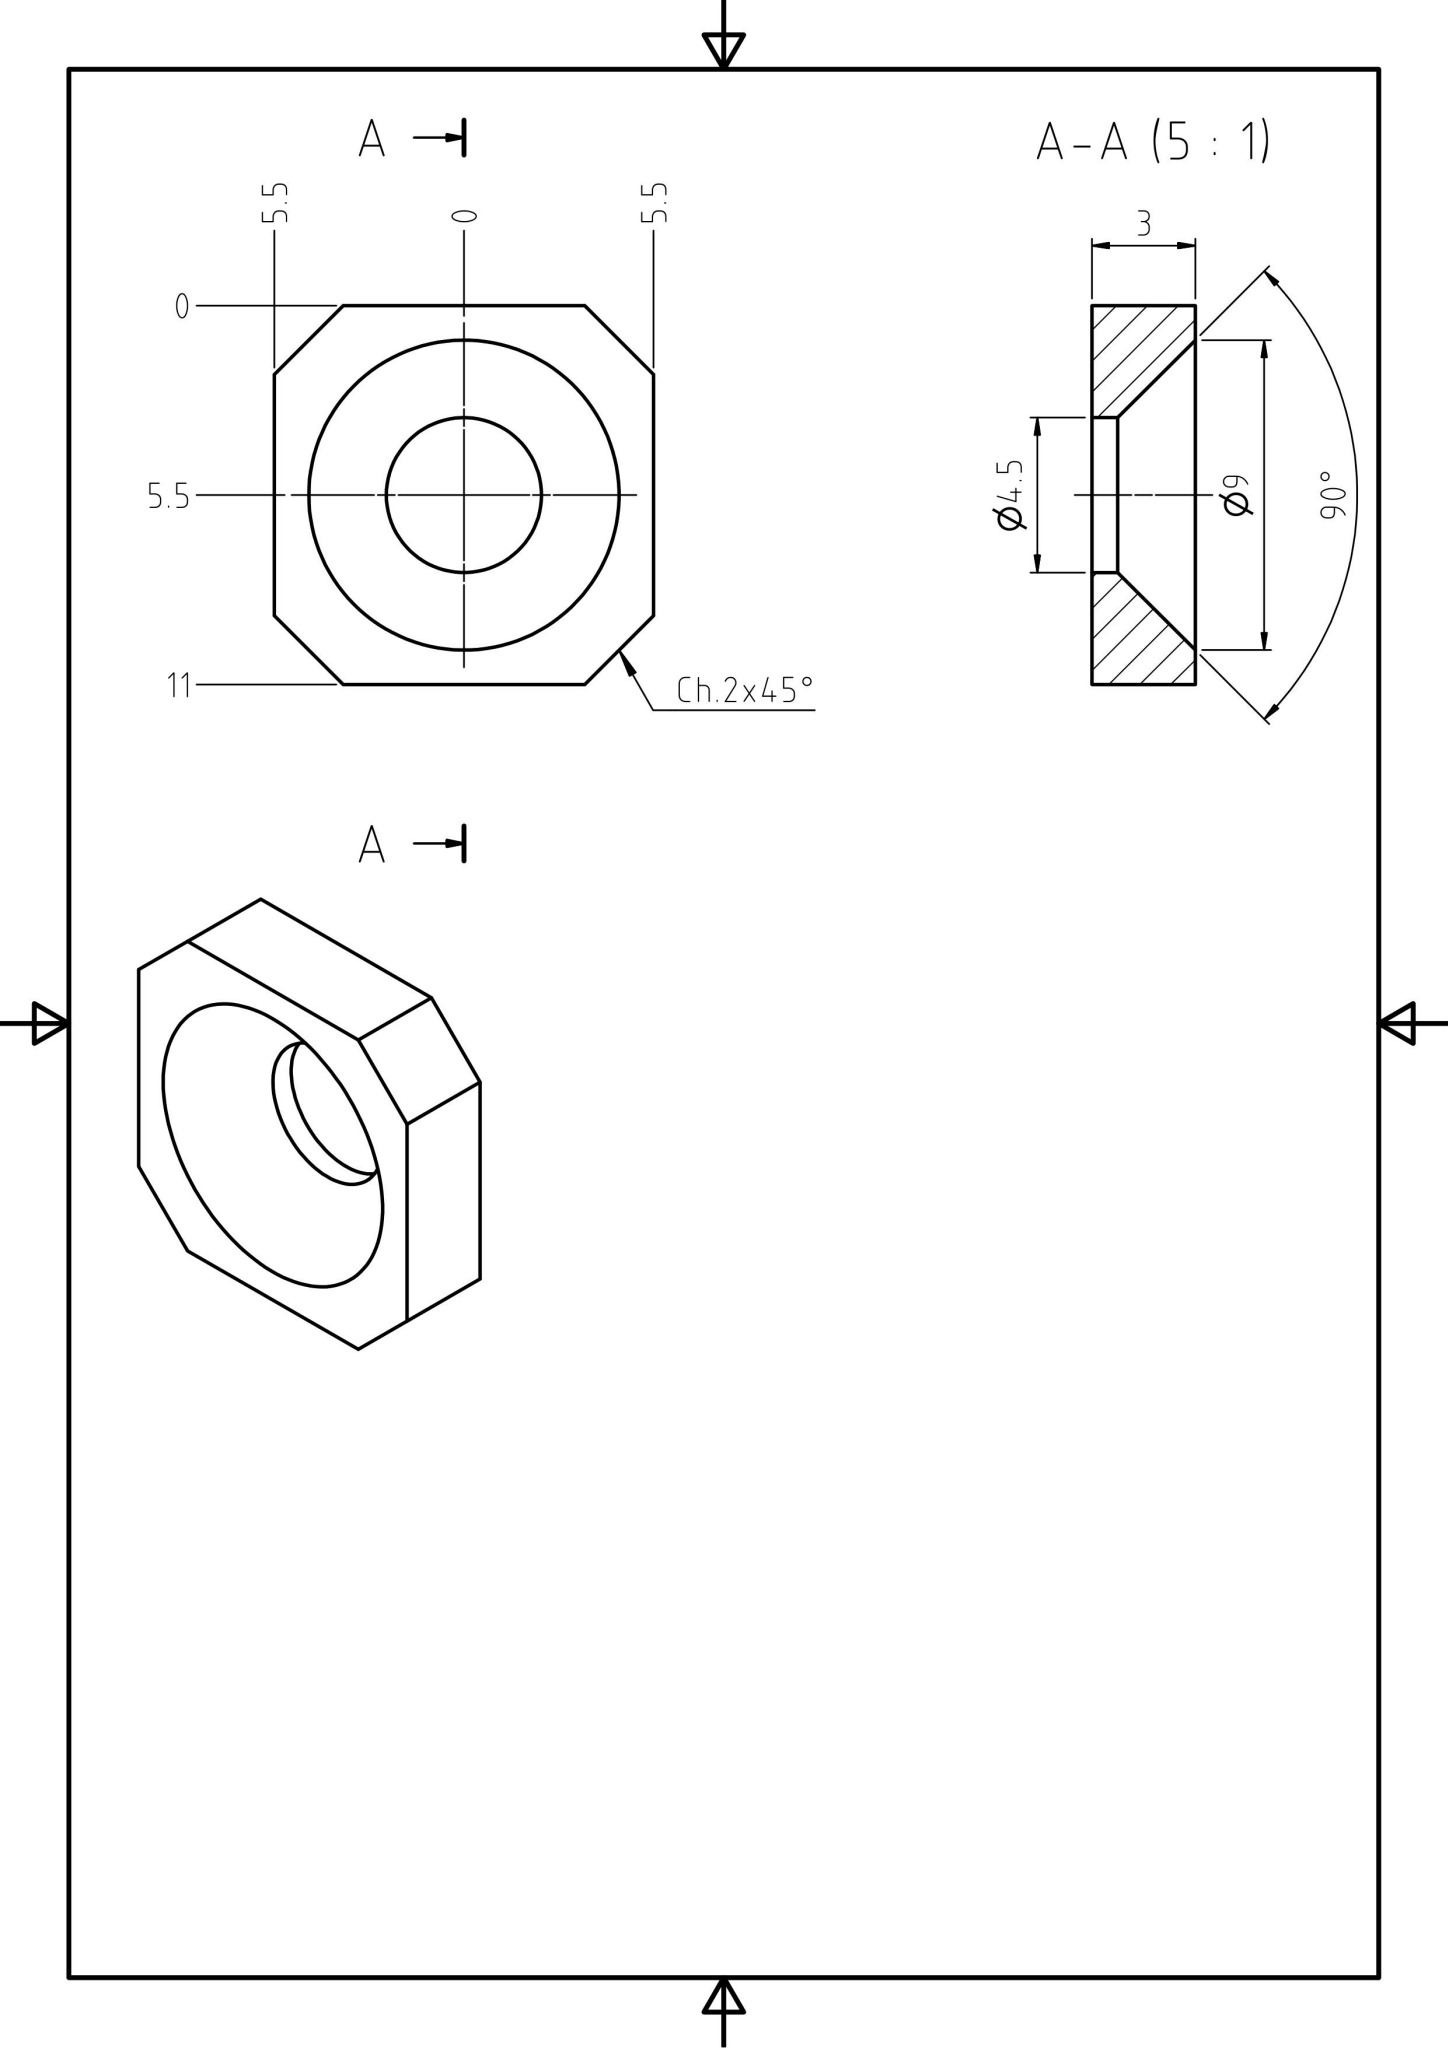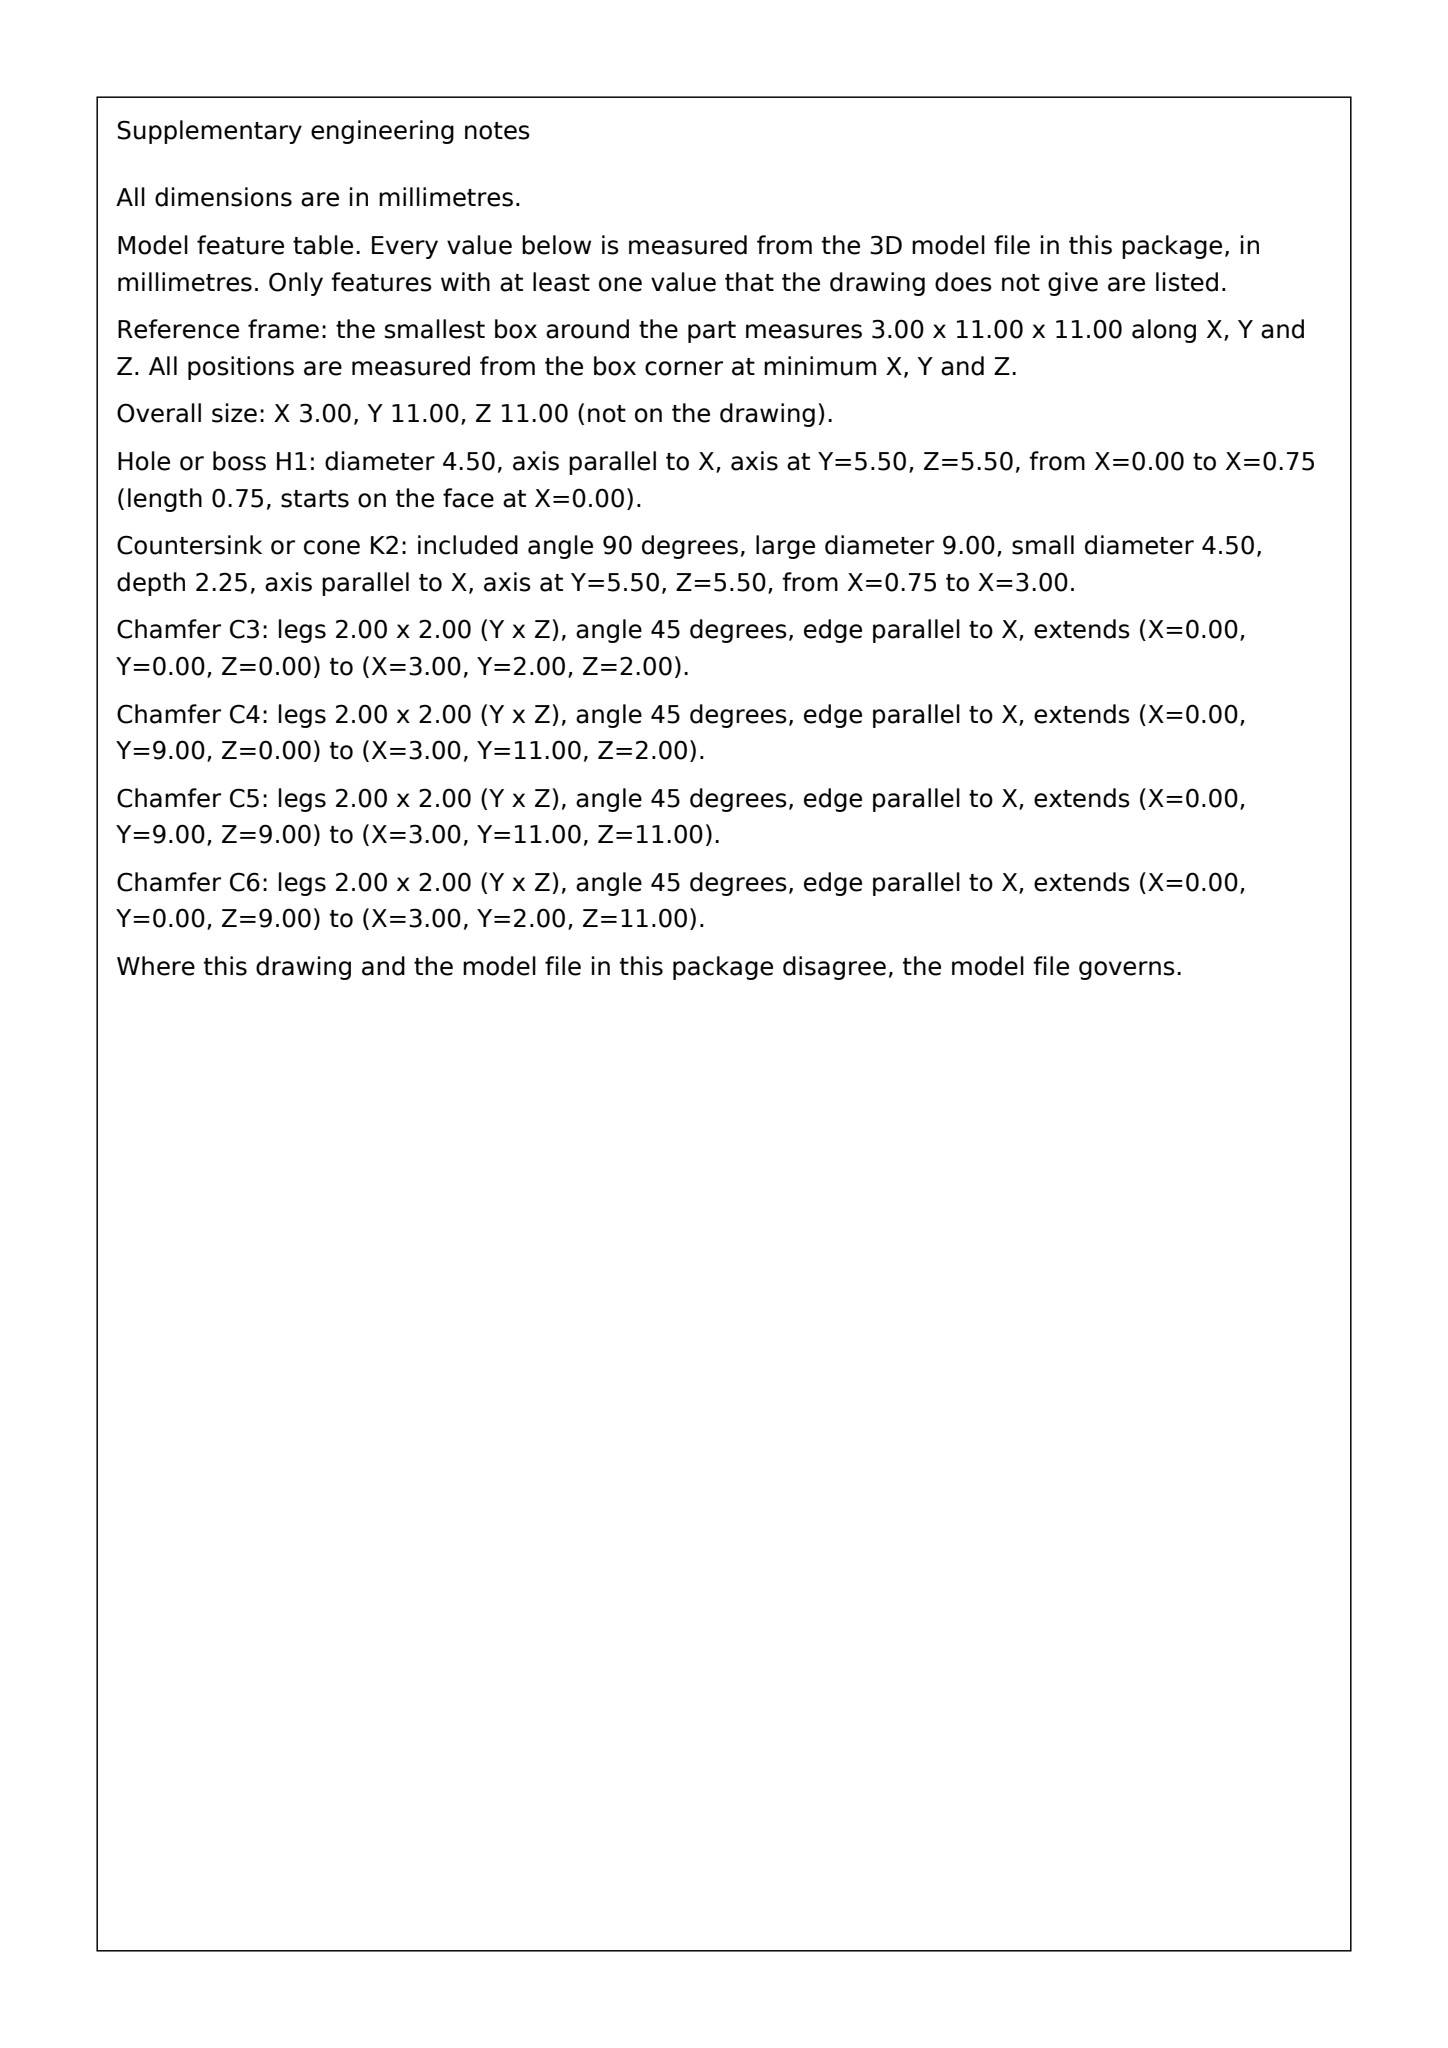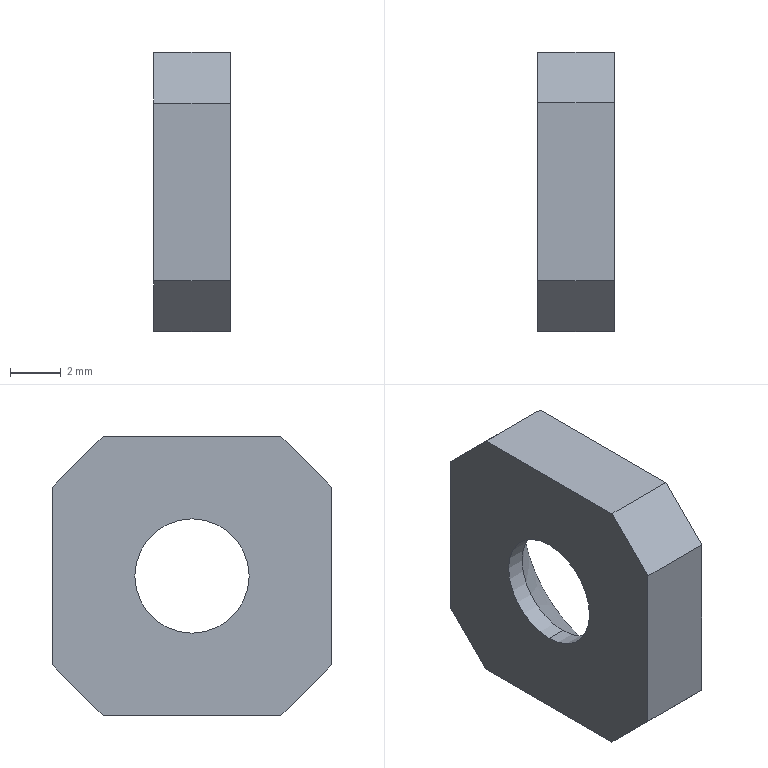Part | SolidWorks | mm | 1 solid | 14 faces | box 3 x 11 x 11 mm | volume 244 mm3 | plane 10 | cylinder 2 | cone 2 | commonest cylinder face diameters 4.5 x2
STEP:
#1=CARTESIAN_POINT('',(0.,0.,2.25));
#2=VERTEX_POINT('',#1);
#3=CARTESIAN_POINT('',(0.,0.,-2.25));
#4=VERTEX_POINT('',#3);
#5=CARTESIAN_POINT('',(0.,0.,0.));
#6=DIRECTION('',(1.,0.,0.));
#7=DIRECTION('',(0.,0.,-1.));
#8=AXIS2_PLACEMENT_3D('',#5,#6,#7);
#9=CIRCLE('',#8,2.25);
#10=EDGE_CURVE('',#2,#4,#9,.T.);
#11=ORIENTED_EDGE('',*,*,#10,.F.);
#12=CARTESIAN_POINT('',(0.75,0.,2.25));
#13=VERTEX_POINT('',#12);
#14=CARTESIAN_POINT('',(-12.843,0.,2.25));
#15=DIRECTION('',(1.,0.,0.));
#16=VECTOR('',#15,1000.);
#17=LINE('',#14,#16);
#18=EDGE_CURVE('',#2,#13,#17,.T.);
#19=ORIENTED_EDGE('',*,*,#18,.T.);
#20=CARTESIAN_POINT('',(0.75,0.,-2.25));
#21=VERTEX_POINT('',#20);
#22=CARTESIAN_POINT('',(0.75,0.,0.));
#23=DIRECTION('',(1.,0.,0.));
#24=DIRECTION('',(0.,0.,-1.));
#25=AXIS2_PLACEMENT_3D('',#22,#23,#24);
#26=CIRCLE('',#25,2.25);
#27=EDGE_CURVE('',#13,#21,#26,.T.);
#28=ORIENTED_EDGE('',*,*,#27,.T.);
#29=CARTESIAN_POINT('',(-12.843,0.,-2.25));
#30=DIRECTION('',(1.,0.,0.));
#31=VECTOR('',#30,1000.);
#32=LINE('',#29,#31);
#33=EDGE_CURVE('',#4,#21,#32,.T.);
#34=ORIENTED_EDGE('',*,*,#33,.F.);
#35=EDGE_LOOP('',(#11,#19,#28,#34));
#36=FACE_OUTER_BOUND('',#35,.T.);
#37=CARTESIAN_POINT('',(-12.843,0.,0.));
#38=DIRECTION('',(1.,0.,0.));
#39=DIRECTION('',(0.,0.,-1.));
#40=AXIS2_PLACEMENT_3D('',#37,#38,#39);
#41=CYLINDRICAL_SURFACE('',#40,2.25);
#42=ADVANCED_FACE('',(#36),#41,.F.);
#43=ORIENTED_EDGE('',*,*,#27,.F.);
#44=CARTESIAN_POINT('',(3.,0.,4.5));
#45=VERTEX_POINT('',#44);
#46=CARTESIAN_POINT('',(1.875,0.,3.375));
#47=DIRECTION('',(0.7071,0.,0.7071));
#48=VECTOR('',#47,1000.);
#49=LINE('',#46,#48);
#50=EDGE_CURVE('',#13,#45,#49,.T.);
#51=ORIENTED_EDGE('',*,*,#50,.T.);
#52=CARTESIAN_POINT('',(3.,0.,-4.5));
#53=VERTEX_POINT('',#52);
#54=CARTESIAN_POINT('',(3.,0.,0.));
#55=DIRECTION('',(-1.,0.,0.));
#56=DIRECTION('',(0.,0.,-1.));
#57=AXIS2_PLACEMENT_3D('',#54,#55,#56);
#58=CIRCLE('',#57,4.5);
#59=EDGE_CURVE('',#53,#45,#58,.T.);
#60=ORIENTED_EDGE('',*,*,#59,.F.);
#61=CARTESIAN_POINT('',(1.875,0.,-3.375));
#62=DIRECTION('',(0.7071,0.,-0.7071));
#63=VECTOR('',#62,1000.);
#64=LINE('',#61,#63);
#65=EDGE_CURVE('',#21,#53,#64,.T.);
#66=ORIENTED_EDGE('',*,*,#65,.F.);
#67=EDGE_LOOP('',(#43,#51,#60,#66));
#68=FACE_OUTER_BOUND('',#67,.T.);
#69=CARTESIAN_POINT('',(1.875,0.,0.));
#70=DIRECTION('',(1.,0.,0.));
#71=DIRECTION('',(0.,0.,-1.));
#72=AXIS2_PLACEMENT_3D('',#69,#70,#71);
#73=CONICAL_SURFACE('',#72,3.375,0.7854);
#74=ADVANCED_FACE('',(#68),#73,.F.);
#75=CARTESIAN_POINT('',(3.,-3.5,-5.5));
#76=VERTEX_POINT('',#75);
#77=CARTESIAN_POINT('',(3.,-5.5,-3.5));
#78=VERTEX_POINT('',#77);
#79=CARTESIAN_POINT('',(3.,-4.5,-4.5));
#80=DIRECTION('',(0.,-0.7071,0.7071));
#81=VECTOR('',#80,1000.);
#82=LINE('',#79,#81);
#83=EDGE_CURVE('',#76,#78,#82,.T.);
#84=ORIENTED_EDGE('',*,*,#83,.T.);
#85=CARTESIAN_POINT('',(0.,-5.5,-3.5));
#86=VERTEX_POINT('',#85);
#87=CARTESIAN_POINT('',(0.,-5.5,-3.5));
#88=DIRECTION('',(-1.,0.,0.));
#89=VECTOR('',#88,1000.);
#90=LINE('',#87,#89);
#91=EDGE_CURVE('',#78,#86,#90,.T.);
#92=ORIENTED_EDGE('',*,*,#91,.T.);
#93=CARTESIAN_POINT('',(0.,-3.5,-5.5));
#94=VERTEX_POINT('',#93);
#95=CARTESIAN_POINT('',(0.,-4.5,-4.5));
#96=DIRECTION('',(0.,0.7071,-0.7071));
#97=VECTOR('',#96,1000.);
#98=LINE('',#95,#97);
#99=EDGE_CURVE('',#86,#94,#98,.T.);
#100=ORIENTED_EDGE('',*,*,#99,.T.);
#101=CARTESIAN_POINT('',(0.,-3.5,-5.5));
#102=DIRECTION('',(1.,0.,0.));
#103=VECTOR('',#102,1000.);
#104=LINE('',#101,#103);
#105=EDGE_CURVE('',#94,#76,#104,.T.);
#106=ORIENTED_EDGE('',*,*,#105,.T.);
#107=EDGE_LOOP('',(#84,#92,#100,#106));
#108=FACE_OUTER_BOUND('',#107,.T.);
#109=CARTESIAN_POINT('',(0.,-4.5,-4.5));
#110=DIRECTION('',(0.,-0.7071,-0.7071));
#111=DIRECTION('',(0.,-0.7071,0.7071));
#112=AXIS2_PLACEMENT_3D('',#109,#110,#111);
#113=PLANE('',#112);
#114=ADVANCED_FACE('',(#108),#113,.T.);
#115=ORIENTED_EDGE('',*,*,#91,.F.);
#116=CARTESIAN_POINT('',(3.,-5.5,3.5));
#117=VERTEX_POINT('',#116);
#118=CARTESIAN_POINT('',(3.,-5.5,5.5));
#119=DIRECTION('',(0.,0.,-1.));
#120=VECTOR('',#119,1000.);
#121=LINE('',#118,#120);
#122=EDGE_CURVE('',#117,#78,#121,.T.);
#123=ORIENTED_EDGE('',*,*,#122,.F.);
#124=CARTESIAN_POINT('',(0.,-5.5,3.5));
#125=VERTEX_POINT('',#124);
#126=CARTESIAN_POINT('',(0.,-5.5,3.5));
#127=DIRECTION('',(1.,0.,0.));
#128=VECTOR('',#127,1000.);
#129=LINE('',#126,#128);
#130=EDGE_CURVE('',#125,#117,#129,.T.);
#131=ORIENTED_EDGE('',*,*,#130,.F.);
#132=CARTESIAN_POINT('',(0.,-5.5,5.5));
#133=DIRECTION('',(0.,0.,-1.));
#134=VECTOR('',#133,1000.);
#135=LINE('',#132,#134);
#136=EDGE_CURVE('',#125,#86,#135,.T.);
#137=ORIENTED_EDGE('',*,*,#136,.T.);
#138=EDGE_LOOP('',(#115,#123,#131,#137));
#139=FACE_OUTER_BOUND('',#138,.T.);
#140=CARTESIAN_POINT('',(0.,-5.5,5.5));
#141=DIRECTION('',(0.,-1.,0.));
#142=DIRECTION('',(0.,0.,-1.));
#143=AXIS2_PLACEMENT_3D('',#140,#141,#142);
#144=PLANE('',#143);
#145=ADVANCED_FACE('',(#139),#144,.T.);
#146=ORIENTED_EDGE('',*,*,#83,.F.);
#147=CARTESIAN_POINT('',(3.,3.5,-5.5));
#148=VERTEX_POINT('',#147);
#149=CARTESIAN_POINT('',(3.,-5.5,-5.5));
#150=DIRECTION('',(0.,1.,0.));
#151=VECTOR('',#150,1000.);
#152=LINE('',#149,#151);
#153=EDGE_CURVE('',#76,#148,#152,.T.);
#154=ORIENTED_EDGE('',*,*,#153,.T.);
#155=CARTESIAN_POINT('',(3.,5.5,-3.5));
#156=VERTEX_POINT('',#155);
#157=CARTESIAN_POINT('',(3.,4.5,-4.5));
#158=DIRECTION('',(0.,-0.7071,-0.7071));
#159=VECTOR('',#158,1000.);
#160=LINE('',#157,#159);
#161=EDGE_CURVE('',#156,#148,#160,.T.);
#162=ORIENTED_EDGE('',*,*,#161,.F.);
#163=CARTESIAN_POINT('',(3.,5.5,3.5));
#164=VERTEX_POINT('',#163);
#165=CARTESIAN_POINT('',(3.,5.5,-5.5));
#166=DIRECTION('',(0.,0.,1.));
#167=VECTOR('',#166,1000.);
#168=LINE('',#165,#167);
#169=EDGE_CURVE('',#156,#164,#168,.T.);
#170=ORIENTED_EDGE('',*,*,#169,.T.);
#171=CARTESIAN_POINT('',(3.,3.5,5.5));
#172=VERTEX_POINT('',#171);
#173=CARTESIAN_POINT('',(3.,4.5,4.5));
#174=DIRECTION('',(0.,0.7071,-0.7071));
#175=VECTOR('',#174,1000.);
#176=LINE('',#173,#175);
#177=EDGE_CURVE('',#172,#164,#176,.T.);
#178=ORIENTED_EDGE('',*,*,#177,.F.);
#179=CARTESIAN_POINT('',(3.,-3.5,5.5));
#180=VERTEX_POINT('',#179);
#181=CARTESIAN_POINT('',(3.,5.5,5.5));
#182=DIRECTION('',(0.,-1.,0.));
#183=VECTOR('',#182,1000.);
#184=LINE('',#181,#183);
#185=EDGE_CURVE('',#172,#180,#184,.T.);
#186=ORIENTED_EDGE('',*,*,#185,.T.);
#187=CARTESIAN_POINT('',(3.,-4.5,4.5));
#188=DIRECTION('',(0.,0.7071,0.7071));
#189=VECTOR('',#188,1000.);
#190=LINE('',#187,#189);
#191=EDGE_CURVE('',#117,#180,#190,.T.);
#192=ORIENTED_EDGE('',*,*,#191,.F.);
#193=ORIENTED_EDGE('',*,*,#122,.T.);
#194=EDGE_LOOP('',(#146,#154,#162,#170,#178,#186,#192,#193));
#195=FACE_OUTER_BOUND('',#194,.T.);
#196=ORIENTED_EDGE('',*,*,#59,.T.);
#197=CARTESIAN_POINT('',(3.,0.,0.));
#198=DIRECTION('',(-1.,0.,0.));
#199=DIRECTION('',(0.,0.,-1.));
#200=AXIS2_PLACEMENT_3D('',#197,#198,#199);
#201=CIRCLE('',#200,4.5);
#202=EDGE_CURVE('',#45,#53,#201,.T.);
#203=ORIENTED_EDGE('',*,*,#202,.T.);
#204=EDGE_LOOP('',(#196,#203));
#205=FACE_BOUND('',#204,.T.);
#206=CARTESIAN_POINT('',(3.,0.,0.));
#207=DIRECTION('',(1.,0.,0.));
#208=DIRECTION('',(0.,1.,0.));
#209=AXIS2_PLACEMENT_3D('',#206,#207,#208);
#210=PLANE('',#209);
#211=ADVANCED_FACE('',(#195,#205),#210,.T.);
#212=ORIENTED_EDGE('',*,*,#161,.T.);
#213=CARTESIAN_POINT('',(0.,3.5,-5.5));
#214=VERTEX_POINT('',#213);
#215=CARTESIAN_POINT('',(0.,3.5,-5.5));
#216=DIRECTION('',(-1.,0.,0.));
#217=VECTOR('',#216,1000.);
#218=LINE('',#215,#217);
#219=EDGE_CURVE('',#148,#214,#218,.T.);
#220=ORIENTED_EDGE('',*,*,#219,.T.);
#221=CARTESIAN_POINT('',(0.,5.5,-3.5));
#222=VERTEX_POINT('',#221);
#223=CARTESIAN_POINT('',(0.,4.5,-4.5));
#224=DIRECTION('',(0.,0.7071,0.7071));
#225=VECTOR('',#224,1000.);
#226=LINE('',#223,#225);
#227=EDGE_CURVE('',#214,#222,#226,.T.);
#228=ORIENTED_EDGE('',*,*,#227,.T.);
#229=CARTESIAN_POINT('',(0.,5.5,-3.5));
#230=DIRECTION('',(1.,0.,0.));
#231=VECTOR('',#230,1000.);
#232=LINE('',#229,#231);
#233=EDGE_CURVE('',#222,#156,#232,.T.);
#234=ORIENTED_EDGE('',*,*,#233,.T.);
#235=EDGE_LOOP('',(#212,#220,#228,#234));
#236=FACE_OUTER_BOUND('',#235,.T.);
#237=CARTESIAN_POINT('',(0.,4.5,-4.5));
#238=DIRECTION('',(0.,0.7071,-0.7071));
#239=DIRECTION('',(-1.,0.,0.));
#240=AXIS2_PLACEMENT_3D('',#237,#238,#239);
#241=PLANE('',#240);
#242=ADVANCED_FACE('',(#236),#241,.T.);
#243=ORIENTED_EDGE('',*,*,#233,.F.);
#244=CARTESIAN_POINT('',(0.,5.5,3.5));
#245=VERTEX_POINT('',#244);
#246=CARTESIAN_POINT('',(0.,5.5,-5.5));
#247=DIRECTION('',(0.,0.,1.));
#248=VECTOR('',#247,1000.);
#249=LINE('',#246,#248);
#250=EDGE_CURVE('',#222,#245,#249,.T.);
#251=ORIENTED_EDGE('',*,*,#250,.T.);
#252=CARTESIAN_POINT('',(0.,5.5,3.5));
#253=DIRECTION('',(-1.,0.,0.));
#254=VECTOR('',#253,1000.);
#255=LINE('',#252,#254);
#256=EDGE_CURVE('',#164,#245,#255,.T.);
#257=ORIENTED_EDGE('',*,*,#256,.F.);
#258=ORIENTED_EDGE('',*,*,#169,.F.);
#259=EDGE_LOOP('',(#243,#251,#257,#258));
#260=FACE_OUTER_BOUND('',#259,.T.);
#261=CARTESIAN_POINT('',(0.,5.5,-5.5));
#262=DIRECTION('',(0.,1.,0.));
#263=DIRECTION('',(1.,0.,0.));
#264=AXIS2_PLACEMENT_3D('',#261,#262,#263);
#265=PLANE('',#264);
#266=ADVANCED_FACE('',(#260),#265,.T.);
#267=ORIENTED_EDGE('',*,*,#177,.T.);
#268=ORIENTED_EDGE('',*,*,#256,.T.);
#269=CARTESIAN_POINT('',(0.,3.5,5.5));
#270=VERTEX_POINT('',#269);
#271=CARTESIAN_POINT('',(0.,4.5,4.5));
#272=DIRECTION('',(0.,-0.7071,0.7071));
#273=VECTOR('',#272,1000.);
#274=LINE('',#271,#273);
#275=EDGE_CURVE('',#245,#270,#274,.T.);
#276=ORIENTED_EDGE('',*,*,#275,.T.);
#277=CARTESIAN_POINT('',(0.,3.5,5.5));
#278=DIRECTION('',(1.,0.,0.));
#279=VECTOR('',#278,1000.);
#280=LINE('',#277,#279);
#281=EDGE_CURVE('',#270,#172,#280,.T.);
#282=ORIENTED_EDGE('',*,*,#281,.T.);
#283=EDGE_LOOP('',(#267,#268,#276,#282));
#284=FACE_OUTER_BOUND('',#283,.T.);
#285=CARTESIAN_POINT('',(0.,4.5,4.5));
#286=DIRECTION('',(0.,0.7071,0.7071));
#287=DIRECTION('',(1.,0.,0.));
#288=AXIS2_PLACEMENT_3D('',#285,#286,#287);
#289=PLANE('',#288);
#290=ADVANCED_FACE('',(#284),#289,.T.);
#291=ORIENTED_EDGE('',*,*,#191,.T.);
#292=CARTESIAN_POINT('',(0.,-3.5,5.5));
#293=VERTEX_POINT('',#292);
#294=CARTESIAN_POINT('',(0.,-3.5,5.5));
#295=DIRECTION('',(-1.,0.,0.));
#296=VECTOR('',#295,1000.);
#297=LINE('',#294,#296);
#298=EDGE_CURVE('',#180,#293,#297,.T.);
#299=ORIENTED_EDGE('',*,*,#298,.T.);
#300=CARTESIAN_POINT('',(0.,-4.5,4.5));
#301=DIRECTION('',(0.,-0.7071,-0.7071));
#302=VECTOR('',#301,1000.);
#303=LINE('',#300,#302);
#304=EDGE_CURVE('',#293,#125,#303,.T.);
#305=ORIENTED_EDGE('',*,*,#304,.T.);
#306=ORIENTED_EDGE('',*,*,#130,.T.);
#307=EDGE_LOOP('',(#291,#299,#305,#306));
#308=FACE_OUTER_BOUND('',#307,.T.);
#309=CARTESIAN_POINT('',(0.,-4.5,4.5));
#310=DIRECTION('',(0.,-0.7071,0.7071));
#311=DIRECTION('',(-1.,0.,0.));
#312=AXIS2_PLACEMENT_3D('',#309,#310,#311);
#313=PLANE('',#312);
#314=ADVANCED_FACE('',(#308),#313,.T.);
#315=ORIENTED_EDGE('',*,*,#50,.F.);
#316=CARTESIAN_POINT('',(0.75,0.,0.));
#317=DIRECTION('',(1.,0.,0.));
#318=DIRECTION('',(0.,0.,-1.));
#319=AXIS2_PLACEMENT_3D('',#316,#317,#318);
#320=CIRCLE('',#319,2.25);
#321=EDGE_CURVE('',#21,#13,#320,.T.);
#322=ORIENTED_EDGE('',*,*,#321,.F.);
#323=ORIENTED_EDGE('',*,*,#65,.T.);
#324=ORIENTED_EDGE('',*,*,#202,.F.);
#325=EDGE_LOOP('',(#315,#322,#323,#324));
#326=FACE_OUTER_BOUND('',#325,.T.);
#327=CARTESIAN_POINT('',(1.875,0.,0.));
#328=DIRECTION('',(1.,0.,0.));
#329=DIRECTION('',(0.,0.,-1.));
#330=AXIS2_PLACEMENT_3D('',#327,#328,#329);
#331=CONICAL_SURFACE('',#330,3.375,0.7854);
#332=ADVANCED_FACE('',(#326),#331,.F.);
#333=ORIENTED_EDGE('',*,*,#18,.F.);
#334=CARTESIAN_POINT('',(0.,0.,0.));
#335=DIRECTION('',(1.,0.,0.));
#336=DIRECTION('',(0.,0.,-1.));
#337=AXIS2_PLACEMENT_3D('',#334,#335,#336);
#338=CIRCLE('',#337,2.25);
#339=EDGE_CURVE('',#4,#2,#338,.T.);
#340=ORIENTED_EDGE('',*,*,#339,.F.);
#341=ORIENTED_EDGE('',*,*,#33,.T.);
#342=ORIENTED_EDGE('',*,*,#321,.T.);
#343=EDGE_LOOP('',(#333,#340,#341,#342));
#344=FACE_OUTER_BOUND('',#343,.T.);
#345=CARTESIAN_POINT('',(-12.843,0.,0.));
#346=DIRECTION('',(1.,0.,0.));
#347=DIRECTION('',(0.,0.,-1.));
#348=AXIS2_PLACEMENT_3D('',#345,#346,#347);
#349=CYLINDRICAL_SURFACE('',#348,2.25);
#350=ADVANCED_FACE('',(#344),#349,.F.);
#351=ORIENTED_EDGE('',*,*,#281,.F.);
#352=CARTESIAN_POINT('',(0.,5.5,5.5));
#353=DIRECTION('',(0.,-1.,0.));
#354=VECTOR('',#353,1000.);
#355=LINE('',#352,#354);
#356=EDGE_CURVE('',#270,#293,#355,.T.);
#357=ORIENTED_EDGE('',*,*,#356,.T.);
#358=ORIENTED_EDGE('',*,*,#298,.F.);
#359=ORIENTED_EDGE('',*,*,#185,.F.);
#360=EDGE_LOOP('',(#351,#357,#358,#359));
#361=FACE_OUTER_BOUND('',#360,.T.);
#362=CARTESIAN_POINT('',(0.,5.5,5.5));
#363=DIRECTION('',(0.,0.,1.));
#364=DIRECTION('',(1.,0.,0.));
#365=AXIS2_PLACEMENT_3D('',#362,#363,#364);
#366=PLANE('',#365);
#367=ADVANCED_FACE('',(#361),#366,.T.);
#368=ORIENTED_EDGE('',*,*,#105,.F.);
#369=CARTESIAN_POINT('',(0.,-5.5,-5.5));
#370=DIRECTION('',(0.,1.,0.));
#371=VECTOR('',#370,1000.);
#372=LINE('',#369,#371);
#373=EDGE_CURVE('',#94,#214,#372,.T.);
#374=ORIENTED_EDGE('',*,*,#373,.T.);
#375=ORIENTED_EDGE('',*,*,#219,.F.);
#376=ORIENTED_EDGE('',*,*,#153,.F.);
#377=EDGE_LOOP('',(#368,#374,#375,#376));
#378=FACE_OUTER_BOUND('',#377,.T.);
#379=CARTESIAN_POINT('',(0.,-5.5,-5.5));
#380=DIRECTION('',(0.,0.,-1.));
#381=DIRECTION('',(0.,-1.,0.));
#382=AXIS2_PLACEMENT_3D('',#379,#380,#381);
#383=PLANE('',#382);
#384=ADVANCED_FACE('',(#378),#383,.T.);
#385=ORIENTED_EDGE('',*,*,#99,.F.);
#386=ORIENTED_EDGE('',*,*,#136,.F.);
#387=ORIENTED_EDGE('',*,*,#304,.F.);
#388=ORIENTED_EDGE('',*,*,#356,.F.);
#389=ORIENTED_EDGE('',*,*,#275,.F.);
#390=ORIENTED_EDGE('',*,*,#250,.F.);
#391=ORIENTED_EDGE('',*,*,#227,.F.);
#392=ORIENTED_EDGE('',*,*,#373,.F.);
#393=EDGE_LOOP('',(#385,#386,#387,#388,#389,#390,#391,#392));
#394=FACE_OUTER_BOUND('',#393,.T.);
#395=ORIENTED_EDGE('',*,*,#339,.T.);
#396=ORIENTED_EDGE('',*,*,#10,.T.);
#397=EDGE_LOOP('',(#395,#396));
#398=FACE_BOUND('',#397,.T.);
#399=CARTESIAN_POINT('',(0.,0.,0.));
#400=DIRECTION('',(1.,0.,0.));
#401=DIRECTION('',(0.,1.,0.));
#402=AXIS2_PLACEMENT_3D('',#399,#400,#401);
#403=PLANE('',#402);
#404=ADVANCED_FACE('',(#394,#398),#403,.F.);
#405=CLOSED_SHELL('',(#42,#74,#114,#145,#211,#242,#266,#290,#314,#332,#350,#367,#384,#404));
#406=MANIFOLD_SOLID_BREP('',#405);
#407=CARTESIAN_POINT('',(0.,0.,0.));
#408=DIRECTION('',(0.,0.,1.));
#409=DIRECTION('',(1.,0.,0.));
#410=AXIS2_PLACEMENT_3D('',#407,#408,#409);
#411=(LENGTH_UNIT()NAMED_UNIT(*)SI_UNIT(.MILLI.,.METRE.));
#412=UNCERTAINTY_MEASURE_WITH_UNIT(LENGTH_MEASURE(0.00001),#411,'','');
#413=(NAMED_UNIT(*)PLANE_ANGLE_UNIT()SI_UNIT($,.RADIAN.));
#414=(NAMED_UNIT(*)SI_UNIT($,.STERADIAN.)SOLID_ANGLE_UNIT());
#415=(GEOMETRIC_REPRESENTATION_CONTEXT(3)GLOBAL_UNCERTAINTY_ASSIGNED_CONTEXT((#412))GLOBAL_UNIT_ASSIGNED_CONTEXT((#411,#413,#414))REPRESENTATION_CONTEXT('',''));
#416=ADVANCED_BREP_SHAPE_REPRESENTATION('',(#406,#410),#415);